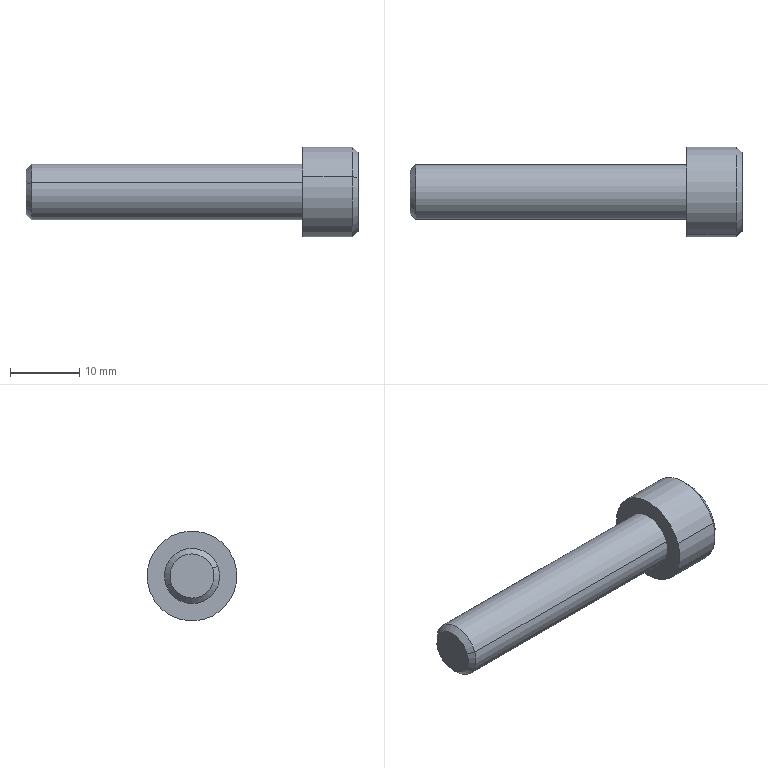Component | SolidWorks | LD101-02-HexagonScrew-M8X40-2-2 | 1 solid | 25 faces | box 48 x 13 x 13 mm | volume 2920 mm3 | plane 15 | cone 6 | cylinder 4 | commonest cylinder face diameters 13 x2 8 x2
STEP:
#1=COLOUR_RGB('',0.7922,0.8196,0.9333);
#2=FILL_AREA_STYLE_COLOUR('',#1);
#3=FILL_AREA_STYLE('',(#2));
#4=SURFACE_STYLE_FILL_AREA(#3);
#5=SURFACE_SIDE_STYLE('',(#4));
#6=SURFACE_STYLE_USAGE(.BOTH.,#5);
#7=PRESENTATION_STYLE_ASSIGNMENT((#6));
#8=CARTESIAN_POINT('',(13.374,-8.5,0.2505));
#9=VERTEX_POINT('',#8);
#10=CARTESIAN_POINT('',(13.374,-8.264,0.1634));
#11=VERTEX_POINT('',#10);
#12=CARTESIAN_POINT('',(13.374,-8.382,0.207));
#13=DIRECTION('',(-1.,0.,0.));
#14=DIRECTION('',(0.,-0.9384,0.3455));
#15=AXIS2_PLACEMENT_3D('',#12,#13,#14);
#16=CIRCLE('',#15,0.126);
#17=EDGE_CURVE('',#9,#11,#16,.T.);
#18=ORIENTED_EDGE('',*,*,#17,.F.);
#19=CARTESIAN_POINT('',(13.406,-8.53,0.2614));
#20=VERTEX_POINT('',#19);
#21=CARTESIAN_POINT('',(13.374,-8.5,0.2505));
#22=DIRECTION('',(0.7071,-0.6636,0.2443));
#23=VECTOR('',#22,39.37);
#24=LINE('',#21,#23);
#25=EDGE_CURVE('',#9,#20,#24,.T.);
#26=ORIENTED_EDGE('',*,*,#25,.T.);
#27=CARTESIAN_POINT('',(13.406,-8.234,0.1525));
#28=VERTEX_POINT('',#27);
#29=CARTESIAN_POINT('',(13.406,-8.382,0.207));
#30=DIRECTION('',(1.,-0.,-0.));
#31=DIRECTION('',(0.,-0.9384,0.3455));
#32=AXIS2_PLACEMENT_3D('',#29,#30,#31);
#33=CIRCLE('',#32,0.1575);
#34=EDGE_CURVE('',#28,#20,#33,.T.);
#35=ORIENTED_EDGE('',*,*,#34,.F.);
#36=CARTESIAN_POINT('',(13.374,-8.264,0.1634));
#37=DIRECTION('',(0.7071,0.6636,-0.2443));
#38=VECTOR('',#37,39.37);
#39=LINE('',#36,#38);
#40=EDGE_CURVE('',#11,#28,#39,.T.);
#41=ORIENTED_EDGE('',*,*,#40,.F.);
#42=EDGE_LOOP('',(#18,#26,#35,#41));
#43=FACE_OUTER_BOUND('',#42,.T.);
#44=CARTESIAN_POINT('',(13.374,-8.382,0.207));
#45=DIRECTION('',(1.,-0.,-0.));
#46=DIRECTION('',(0.,0.9384,-0.3455));
#47=AXIS2_PLACEMENT_3D('',#44,#45,#46);
#48=CONICAL_SURFACE('',#47,0.126,0.7854);
#49=ADVANCED_FACE('',(#43),#48,.T.);
#50=CARTESIAN_POINT('',(15.233,-8.622,0.2954));
#51=VERTEX_POINT('',#50);
#52=CARTESIAN_POINT('',(15.233,-8.142,0.1185));
#53=VERTEX_POINT('',#52);
#54=CARTESIAN_POINT('',(15.233,-8.382,0.207));
#55=DIRECTION('',(-1.,0.,0.));
#56=DIRECTION('',(0.,-0.9384,0.3455));
#57=AXIS2_PLACEMENT_3D('',#54,#55,#56);
#58=CIRCLE('',#57,0.2559);
#59=EDGE_CURVE('',#51,#53,#58,.T.);
#60=ORIENTED_EDGE('',*,*,#59,.T.);
#61=CARTESIAN_POINT('',(14.949,-8.142,0.1185));
#62=VERTEX_POINT('',#61);
#63=CARTESIAN_POINT('',(15.091,-8.142,0.1185));
#64=DIRECTION('',(-1.,0.,0.));
#65=VECTOR('',#64,39.37);
#66=LINE('',#63,#65);
#67=EDGE_CURVE('',#53,#62,#66,.T.);
#68=ORIENTED_EDGE('',*,*,#67,.T.);
#69=CARTESIAN_POINT('',(14.949,-8.622,0.2954));
#70=VERTEX_POINT('',#69);
#71=CARTESIAN_POINT('',(14.949,-8.382,0.207));
#72=DIRECTION('',(1.,-0.,-0.));
#73=DIRECTION('',(0.,-0.9384,0.3455));
#74=AXIS2_PLACEMENT_3D('',#71,#72,#73);
#75=CIRCLE('',#74,0.2559);
#76=EDGE_CURVE('',#62,#70,#75,.T.);
#77=ORIENTED_EDGE('',*,*,#76,.T.);
#78=CARTESIAN_POINT('',(15.091,-8.622,0.2954));
#79=DIRECTION('',(-1.,0.,0.));
#80=VECTOR('',#79,39.37);
#81=LINE('',#78,#80);
#82=EDGE_CURVE('',#51,#70,#81,.T.);
#83=ORIENTED_EDGE('',*,*,#82,.F.);
#84=EDGE_LOOP('',(#60,#68,#77,#83));
#85=FACE_OUTER_BOUND('',#84,.T.);
#86=CARTESIAN_POINT('',(15.091,-8.382,0.207));
#87=DIRECTION('',(-1.,0.,0.));
#88=DIRECTION('',(0.,-0.9384,0.3455));
#89=AXIS2_PLACEMENT_3D('',#86,#87,#88);
#90=CYLINDRICAL_SURFACE('',#89,0.2559);
#91=ADVANCED_FACE('',(#85),#90,.T.);
#92=CARTESIAN_POINT('',(15.264,-8.592,0.2845));
#93=VERTEX_POINT('',#92);
#94=CARTESIAN_POINT('',(15.264,-8.171,0.1294));
#95=VERTEX_POINT('',#94);
#96=CARTESIAN_POINT('',(15.264,-8.382,0.207));
#97=DIRECTION('',(-1.,0.,0.));
#98=DIRECTION('',(0.,-0.9384,0.3455));
#99=AXIS2_PLACEMENT_3D('',#96,#97,#98);
#100=CIRCLE('',#99,0.2244);
#101=EDGE_CURVE('',#93,#95,#100,.T.);
#102=ORIENTED_EDGE('',*,*,#101,.T.);
#103=CARTESIAN_POINT('',(15.233,-8.142,0.1185));
#104=DIRECTION('',(-0.7071,0.6636,-0.2443));
#105=VECTOR('',#104,39.37);
#106=LINE('',#103,#105);
#107=EDGE_CURVE('',#95,#53,#106,.T.);
#108=ORIENTED_EDGE('',*,*,#107,.T.);
#109=ORIENTED_EDGE('',*,*,#59,.F.);
#110=CARTESIAN_POINT('',(15.233,-8.622,0.2954));
#111=DIRECTION('',(-0.7071,-0.6636,0.2443));
#112=VECTOR('',#111,39.37);
#113=LINE('',#110,#112);
#114=EDGE_CURVE('',#93,#51,#113,.T.);
#115=ORIENTED_EDGE('',*,*,#114,.F.);
#116=EDGE_LOOP('',(#102,#108,#109,#115));
#117=FACE_OUTER_BOUND('',#116,.T.);
#118=CARTESIAN_POINT('',(15.233,-8.382,0.207));
#119=DIRECTION('',(-1.,0.,0.));
#120=DIRECTION('',(0.,-0.9384,0.3455));
#121=AXIS2_PLACEMENT_3D('',#118,#119,#120);
#122=CONICAL_SURFACE('',#121,0.2559,0.7854);
#123=ADVANCED_FACE('',(#117),#122,.T.);
#124=CARTESIAN_POINT('',(14.949,-8.234,0.1525));
#125=VERTEX_POINT('',#124);
#126=CARTESIAN_POINT('',(14.949,-8.53,0.2614));
#127=VERTEX_POINT('',#126);
#128=CARTESIAN_POINT('',(14.949,-8.382,0.207));
#129=DIRECTION('',(1.,-0.,-0.));
#130=DIRECTION('',(0.,-0.9384,0.3455));
#131=AXIS2_PLACEMENT_3D('',#128,#129,#130);
#132=CIRCLE('',#131,0.1575);
#133=EDGE_CURVE('',#125,#127,#132,.T.);
#134=ORIENTED_EDGE('',*,*,#133,.F.);
#135=CARTESIAN_POINT('',(14.767,-8.234,0.1525));
#136=DIRECTION('',(-1.,0.,0.));
#137=VECTOR('',#136,39.37);
#138=LINE('',#135,#137);
#139=EDGE_CURVE('',#125,#28,#138,.T.);
#140=ORIENTED_EDGE('',*,*,#139,.T.);
#141=ORIENTED_EDGE('',*,*,#34,.T.);
#142=CARTESIAN_POINT('',(14.767,-8.53,0.2614));
#143=DIRECTION('',(-1.,0.,0.));
#144=VECTOR('',#143,39.37);
#145=LINE('',#142,#144);
#146=EDGE_CURVE('',#127,#20,#145,.T.);
#147=ORIENTED_EDGE('',*,*,#146,.F.);
#148=EDGE_LOOP('',(#134,#140,#141,#147));
#149=FACE_OUTER_BOUND('',#148,.T.);
#150=CARTESIAN_POINT('',(14.767,-8.382,0.207));
#151=DIRECTION('',(-1.,0.,0.));
#152=DIRECTION('',(0.,-0.9384,0.3455));
#153=AXIS2_PLACEMENT_3D('',#150,#151,#152);
#154=CYLINDRICAL_SURFACE('',#153,0.1575);
#155=ADVANCED_FACE('',(#149),#154,.T.);
#156=CARTESIAN_POINT('',(15.075,-8.382,0.207));
#157=VERTEX_POINT('',#156);
#158=CARTESIAN_POINT('',(15.107,-8.271,0.1661));
#159=VERTEX_POINT('',#158);
#160=CARTESIAN_POINT('',(15.107,-8.271,0.1661));
#161=DIRECTION('',(0.2588,0.9064,-0.3338));
#162=VECTOR('',#161,39.37);
#163=LINE('',#160,#162);
#164=EDGE_CURVE('',#157,#159,#163,.T.);
#165=ORIENTED_EDGE('',*,*,#164,.F.);
#166=CARTESIAN_POINT('',(15.107,-8.493,0.2478));
#167=VERTEX_POINT('',#166);
#168=CARTESIAN_POINT('',(15.107,-8.493,0.2478));
#169=DIRECTION('',(0.2588,-0.9064,0.3338));
#170=VECTOR('',#169,39.37);
#171=LINE('',#168,#170);
#172=EDGE_CURVE('',#157,#167,#171,.T.);
#173=ORIENTED_EDGE('',*,*,#172,.T.);
#174=CARTESIAN_POINT('',(15.107,-8.473,0.1314));
#175=VERTEX_POINT('',#174);
#176=CARTESIAN_POINT('',(15.107,-8.382,0.207));
#177=DIRECTION('',(-1.,0.,0.));
#178=DIRECTION('',(0.,0.9384,-0.3455));
#179=AXIS2_PLACEMENT_3D('',#176,#177,#178);
#180=CIRCLE('',#179,0.1181);
#181=EDGE_CURVE('',#175,#167,#180,.T.);
#182=ORIENTED_EDGE('',*,*,#181,.F.);
#183=CARTESIAN_POINT('',(15.107,-8.362,0.09056));
#184=VERTEX_POINT('',#183);
#185=CARTESIAN_POINT('',(15.107,-8.382,0.207));
#186=DIRECTION('',(-1.,0.,0.));
#187=DIRECTION('',(0.,0.9384,-0.3455));
#188=AXIS2_PLACEMENT_3D('',#185,#186,#187);
#189=CIRCLE('',#188,0.1181);
#190=EDGE_CURVE('',#184,#175,#189,.T.);
#191=ORIENTED_EDGE('',*,*,#190,.F.);
#192=CARTESIAN_POINT('',(15.107,-8.382,0.207));
#193=DIRECTION('',(1.,-0.,-0.));
#194=DIRECTION('',(0.,0.9384,-0.3455));
#195=AXIS2_PLACEMENT_3D('',#192,#193,#194);
#196=CIRCLE('',#195,0.1181);
#197=EDGE_CURVE('',#184,#159,#196,.T.);
#198=ORIENTED_EDGE('',*,*,#197,.T.);
#199=EDGE_LOOP('',(#165,#173,#182,#191,#198));
#200=FACE_OUTER_BOUND('',#199,.T.);
#201=CARTESIAN_POINT('',(15.107,-8.382,0.207));
#202=DIRECTION('',(1.,-0.,-0.));
#203=DIRECTION('',(0.,0.9384,-0.3455));
#204=AXIS2_PLACEMENT_3D('',#201,#202,#203);
#205=CONICAL_SURFACE('',#204,0.1181,1.309);
#206=ADVANCED_FACE('',(#200),#205,.F.);
#207=ORIENTED_EDGE('',*,*,#67,.F.);
#208=CARTESIAN_POINT('',(15.233,-8.382,0.207));
#209=DIRECTION('',(-1.,0.,0.));
#210=DIRECTION('',(0.,-0.9384,0.3455));
#211=AXIS2_PLACEMENT_3D('',#208,#209,#210);
#212=CIRCLE('',#211,0.2559);
#213=EDGE_CURVE('',#53,#51,#212,.T.);
#214=ORIENTED_EDGE('',*,*,#213,.T.);
#215=ORIENTED_EDGE('',*,*,#82,.T.);
#216=CARTESIAN_POINT('',(14.949,-8.382,0.207));
#217=DIRECTION('',(1.,-0.,-0.));
#218=DIRECTION('',(0.,-0.9384,0.3455));
#219=AXIS2_PLACEMENT_3D('',#216,#217,#218);
#220=CIRCLE('',#219,0.2559);
#221=EDGE_CURVE('',#70,#62,#220,.T.);
#222=ORIENTED_EDGE('',*,*,#221,.T.);
#223=EDGE_LOOP('',(#207,#214,#215,#222));
#224=FACE_OUTER_BOUND('',#223,.T.);
#225=CARTESIAN_POINT('',(15.091,-8.382,0.207));
#226=DIRECTION('',(-1.,0.,0.));
#227=DIRECTION('',(0.,-0.9384,0.3455));
#228=AXIS2_PLACEMENT_3D('',#225,#226,#227);
#229=CYLINDRICAL_SURFACE('',#228,0.2559);
#230=ADVANCED_FACE('',(#224),#229,.T.);
#231=ORIENTED_EDGE('',*,*,#107,.F.);
#232=CARTESIAN_POINT('',(15.264,-8.382,0.207));
#233=DIRECTION('',(-1.,0.,0.));
#234=DIRECTION('',(0.,-0.9384,0.3455));
#235=AXIS2_PLACEMENT_3D('',#232,#233,#234);
#236=CIRCLE('',#235,0.2244);
#237=EDGE_CURVE('',#95,#93,#236,.T.);
#238=ORIENTED_EDGE('',*,*,#237,.T.);
#239=ORIENTED_EDGE('',*,*,#114,.T.);
#240=ORIENTED_EDGE('',*,*,#213,.F.);
#241=EDGE_LOOP('',(#231,#238,#239,#240));
#242=FACE_OUTER_BOUND('',#241,.T.);
#243=CARTESIAN_POINT('',(15.233,-8.382,0.207));
#244=DIRECTION('',(-1.,0.,0.));
#245=DIRECTION('',(0.,-0.9384,0.3455));
#246=AXIS2_PLACEMENT_3D('',#243,#244,#245);
#247=CONICAL_SURFACE('',#246,0.2559,0.7854);
#248=ADVANCED_FACE('',(#242),#247,.T.);
#249=CARTESIAN_POINT('',(14.949,-8.382,0.207));
#250=DIRECTION('',(1.,-0.,-0.));
#251=DIRECTION('',(0.,-0.9384,0.3455));
#252=AXIS2_PLACEMENT_3D('',#249,#250,#251);
#253=CIRCLE('',#252,0.1575);
#254=EDGE_CURVE('',#127,#125,#253,.T.);
#255=ORIENTED_EDGE('',*,*,#254,.T.);
#256=ORIENTED_EDGE('',*,*,#133,.T.);
#257=EDGE_LOOP('',(#255,#256));
#258=FACE_BOUND('',#257,.T.);
#259=ORIENTED_EDGE('',*,*,#221,.F.);
#260=ORIENTED_EDGE('',*,*,#76,.F.);
#261=EDGE_LOOP('',(#259,#260));
#262=FACE_OUTER_BOUND('',#261,.T.);
#263=CARTESIAN_POINT('',(14.949,-8.31,0.4009));
#264=DIRECTION('',(-1.,0.,0.));
#265=DIRECTION('',(-0.,-0.9384,0.3455));
#266=AXIS2_PLACEMENT_3D('',#263,#264,#265);
#267=PLANE('',#266);
#268=ADVANCED_FACE('',(#258,#262),#267,.T.);
#269=ORIENTED_EDGE('',*,*,#101,.F.);
#270=ORIENTED_EDGE('',*,*,#237,.F.);
#271=EDGE_LOOP('',(#269,#270));
#272=FACE_OUTER_BOUND('',#271,.T.);
#273=CARTESIAN_POINT('',(15.264,-8.469,0.3118));
#274=VERTEX_POINT('',#273);
#275=CARTESIAN_POINT('',(15.264,-8.335,0.3349));
#276=VERTEX_POINT('',#275);
#277=CARTESIAN_POINT('',(15.264,-8.469,0.3118));
#278=DIRECTION('',(0.,0.9855,0.17));
#279=VECTOR('',#278,39.37);
#280=LINE('',#277,#279);
#281=EDGE_CURVE('',#274,#276,#280,.T.);
#282=ORIENTED_EDGE('',*,*,#281,.T.);
#283=CARTESIAN_POINT('',(15.264,-8.247,0.2301));
#284=VERTEX_POINT('',#283);
#285=CARTESIAN_POINT('',(15.264,-8.335,0.3349));
#286=DIRECTION('',(0.,0.6399,-0.7684));
#287=VECTOR('',#286,39.37);
#288=LINE('',#285,#287);
#289=EDGE_CURVE('',#276,#284,#288,.T.);
#290=ORIENTED_EDGE('',*,*,#289,.T.);
#291=CARTESIAN_POINT('',(15.264,-8.294,0.1022));
#292=VERTEX_POINT('',#291);
#293=CARTESIAN_POINT('',(15.264,-8.232,0.2714));
#294=DIRECTION('',(-0.,-0.3455,-0.9384));
#295=VECTOR('',#294,39.37);
#296=LINE('',#293,#295);
#297=EDGE_CURVE('',#284,#292,#296,.T.);
#298=ORIENTED_EDGE('',*,*,#297,.T.);
#299=CARTESIAN_POINT('',(15.264,-8.429,0.07897));
#300=VERTEX_POINT('',#299);
#301=CARTESIAN_POINT('',(15.264,-8.294,0.1022));
#302=DIRECTION('',(-0.,-0.9855,-0.17));
#303=VECTOR('',#302,39.37);
#304=LINE('',#301,#303);
#305=EDGE_CURVE('',#292,#300,#304,.T.);
#306=ORIENTED_EDGE('',*,*,#305,.T.);
#307=CARTESIAN_POINT('',(15.264,-8.516,0.1838));
#308=VERTEX_POINT('',#307);
#309=CARTESIAN_POINT('',(15.264,-8.429,0.07897));
#310=DIRECTION('',(-0.,-0.6399,0.7684));
#311=VECTOR('',#310,39.37);
#312=LINE('',#309,#311);
#313=EDGE_CURVE('',#300,#308,#312,.T.);
#314=ORIENTED_EDGE('',*,*,#313,.T.);
#315=CARTESIAN_POINT('',(15.264,-8.454,0.3531));
#316=DIRECTION('',(0.,0.3455,0.9384));
#317=VECTOR('',#316,39.37);
#318=LINE('',#315,#317);
#319=EDGE_CURVE('',#308,#274,#318,.T.);
#320=ORIENTED_EDGE('',*,*,#319,.T.);
#321=EDGE_LOOP('',(#282,#290,#298,#306,#314,#320));
#322=FACE_BOUND('',#321,.T.);
#323=CARTESIAN_POINT('',(15.264,-8.343,0.3122));
#324=DIRECTION('',(1.,-0.,-0.));
#325=DIRECTION('',(0.,0.9384,-0.3455));
#326=AXIS2_PLACEMENT_3D('',#323,#324,#325);
#327=PLANE('',#326);
#328=ADVANCED_FACE('',(#272,#322),#327,.T.);
#329=ORIENTED_EDGE('',*,*,#139,.F.);
#330=ORIENTED_EDGE('',*,*,#254,.F.);
#331=ORIENTED_EDGE('',*,*,#146,.T.);
#332=CARTESIAN_POINT('',(13.406,-8.382,0.207));
#333=DIRECTION('',(1.,-0.,-0.));
#334=DIRECTION('',(0.,-0.9384,0.3455));
#335=AXIS2_PLACEMENT_3D('',#332,#333,#334);
#336=CIRCLE('',#335,0.1575);
#337=EDGE_CURVE('',#20,#28,#336,.T.);
#338=ORIENTED_EDGE('',*,*,#337,.T.);
#339=EDGE_LOOP('',(#329,#330,#331,#338));
#340=FACE_OUTER_BOUND('',#339,.T.);
#341=CARTESIAN_POINT('',(14.767,-8.382,0.207));
#342=DIRECTION('',(-1.,0.,0.));
#343=DIRECTION('',(0.,-0.9384,0.3455));
#344=AXIS2_PLACEMENT_3D('',#341,#342,#343);
#345=CYLINDRICAL_SURFACE('',#344,0.1575);
#346=ADVANCED_FACE('',(#340),#345,.T.);
#347=CARTESIAN_POINT('',(15.107,-8.335,0.3349));
#348=VERTEX_POINT('',#347);
#349=CARTESIAN_POINT('',(15.264,-8.335,0.3349));
#350=DIRECTION('',(1.,-0.,-0.));
#351=VECTOR('',#350,39.37);
#352=LINE('',#349,#351);
#353=EDGE_CURVE('',#348,#276,#352,.T.);
#354=ORIENTED_EDGE('',*,*,#353,.F.);
#355=CARTESIAN_POINT('',(15.107,-8.291,0.2825));
#356=VERTEX_POINT('',#355);
#357=CARTESIAN_POINT('',(15.107,-8.247,0.2301));
#358=DIRECTION('',(-0.,-0.6399,0.7684));
#359=VECTOR('',#358,39.37);
#360=LINE('',#357,#359);
#361=EDGE_CURVE('',#356,#348,#360,.T.);
#362=ORIENTED_EDGE('',*,*,#361,.F.);
#363=CARTESIAN_POINT('',(15.107,-8.247,0.2301));
#364=VERTEX_POINT('',#363);
#365=CARTESIAN_POINT('',(15.107,-8.291,0.2825));
#366=DIRECTION('',(0.,0.6399,-0.7684));
#367=VECTOR('',#366,39.37);
#368=LINE('',#365,#367);
#369=EDGE_CURVE('',#356,#364,#368,.T.);
#370=ORIENTED_EDGE('',*,*,#369,.T.);
#371=CARTESIAN_POINT('',(15.264,-8.247,0.2301));
#372=DIRECTION('',(-1.,0.,0.));
#373=VECTOR('',#372,39.37);
#374=LINE('',#371,#373);
#375=EDGE_CURVE('',#284,#364,#374,.T.);
#376=ORIENTED_EDGE('',*,*,#375,.F.);
#377=ORIENTED_EDGE('',*,*,#289,.F.);
#378=EDGE_LOOP('',(#354,#362,#370,#376,#377));
#379=FACE_OUTER_BOUND('',#378,.T.);
#380=CARTESIAN_POINT('',(15.264,-8.247,0.2301));
#381=DIRECTION('',(0.,0.7684,0.6399));
#382=DIRECTION('',(0.,0.6399,-0.7684));
#383=AXIS2_PLACEMENT_3D('',#380,#381,#382);
#384=PLANE('',#383);
#385=ADVANCED_FACE('',(#379),#384,.F.);
#386=CARTESIAN_POINT('',(15.107,-8.469,0.3118));
#387=VERTEX_POINT('',#386);
#388=CARTESIAN_POINT('',(15.264,-8.469,0.3118));
#389=DIRECTION('',(1.,-0.,-0.));
#390=VECTOR('',#389,39.37);
#391=LINE('',#388,#390);
#392=EDGE_CURVE('',#387,#274,#391,.T.);
#393=ORIENTED_EDGE('',*,*,#392,.F.);
#394=CARTESIAN_POINT('',(15.107,-8.402,0.3233));
#395=VERTEX_POINT('',#394);
#396=CARTESIAN_POINT('',(15.107,-8.469,0.3118));
#397=DIRECTION('',(0.,0.9855,0.17));
#398=VECTOR('',#397,39.37);
#399=LINE('',#396,#398);
#400=EDGE_CURVE('',#387,#395,#399,.T.);
#401=ORIENTED_EDGE('',*,*,#400,.T.);
#402=CARTESIAN_POINT('',(15.107,-8.335,0.3349));
#403=DIRECTION('',(-0.,-0.9855,-0.17));
#404=VECTOR('',#403,39.37);
#405=LINE('',#402,#404);
#406=EDGE_CURVE('',#348,#395,#405,.T.);
#407=ORIENTED_EDGE('',*,*,#406,.F.);
#408=ORIENTED_EDGE('',*,*,#353,.T.);
#409=ORIENTED_EDGE('',*,*,#281,.F.);
#410=EDGE_LOOP('',(#393,#401,#407,#408,#409));
#411=FACE_OUTER_BOUND('',#410,.T.);
#412=CARTESIAN_POINT('',(15.264,-8.335,0.3349));
#413=DIRECTION('',(-0.,-0.17,0.9855));
#414=DIRECTION('',(0.,0.9855,0.17));
#415=AXIS2_PLACEMENT_3D('',#412,#413,#414);
#416=PLANE('',#415);
#417=ADVANCED_FACE('',(#411),#416,.F.);
#418=CARTESIAN_POINT('',(15.107,-8.516,0.1838));
#419=VERTEX_POINT('',#418);
#420=CARTESIAN_POINT('',(15.264,-8.516,0.1838));
#421=DIRECTION('',(1.,-0.,-0.));
#422=VECTOR('',#421,39.37);
#423=LINE('',#420,#422);
#424=EDGE_CURVE('',#419,#308,#423,.T.);
#425=ORIENTED_EDGE('',*,*,#424,.F.);
#426=CARTESIAN_POINT('',(15.107,-8.493,0.2478));
#427=DIRECTION('',(0.,0.3455,0.9384));
#428=VECTOR('',#427,39.37);
#429=LINE('',#426,#428);
#430=EDGE_CURVE('',#419,#167,#429,.T.);
#431=ORIENTED_EDGE('',*,*,#430,.T.);
#432=CARTESIAN_POINT('',(15.107,-8.493,0.2478));
#433=DIRECTION('',(0.,0.3455,0.9384));
#434=VECTOR('',#433,39.37);
#435=LINE('',#432,#434);
#436=EDGE_CURVE('',#167,#387,#435,.T.);
#437=ORIENTED_EDGE('',*,*,#436,.T.);
#438=ORIENTED_EDGE('',*,*,#392,.T.);
#439=ORIENTED_EDGE('',*,*,#319,.F.);
#440=EDGE_LOOP('',(#425,#431,#437,#438,#439));
#441=FACE_OUTER_BOUND('',#440,.T.);
#442=CARTESIAN_POINT('',(15.264,-8.469,0.3118));
#443=DIRECTION('',(-0.,-0.9384,0.3455));
#444=DIRECTION('',(1.,-0.,-0.));
#445=AXIS2_PLACEMENT_3D('',#442,#443,#444);
#446=PLANE('',#445);
#447=ADVANCED_FACE('',(#441),#446,.F.);
#448=CARTESIAN_POINT('',(15.107,-8.429,0.07897));
#449=VERTEX_POINT('',#448);
#450=CARTESIAN_POINT('',(15.264,-8.429,0.07897));
#451=DIRECTION('',(1.,-0.,-0.));
#452=VECTOR('',#451,39.37);
#453=LINE('',#450,#452);
#454=EDGE_CURVE('',#449,#300,#453,.T.);
#455=ORIENTED_EDGE('',*,*,#454,.F.);
#456=CARTESIAN_POINT('',(15.107,-8.516,0.1838));
#457=DIRECTION('',(0.,0.6399,-0.7684));
#458=VECTOR('',#457,39.37);
#459=LINE('',#456,#458);
#460=EDGE_CURVE('',#175,#449,#459,.T.);
#461=ORIENTED_EDGE('',*,*,#460,.F.);
#462=CARTESIAN_POINT('',(15.107,-8.473,0.1314));
#463=DIRECTION('',(-0.,-0.6399,0.7684));
#464=VECTOR('',#463,39.37);
#465=LINE('',#462,#464);
#466=EDGE_CURVE('',#175,#419,#465,.T.);
#467=ORIENTED_EDGE('',*,*,#466,.T.);
#468=ORIENTED_EDGE('',*,*,#424,.T.);
#469=ORIENTED_EDGE('',*,*,#313,.F.);
#470=EDGE_LOOP('',(#455,#461,#467,#468,#469));
#471=FACE_OUTER_BOUND('',#470,.T.);
#472=CARTESIAN_POINT('',(15.264,-8.516,0.1838));
#473=DIRECTION('',(-0.,-0.7684,-0.6399));
#474=DIRECTION('',(-0.,-0.6399,0.7684));
#475=AXIS2_PLACEMENT_3D('',#472,#473,#474);
#476=PLANE('',#475);
#477=ADVANCED_FACE('',(#471),#476,.F.);
#478=CARTESIAN_POINT('',(15.107,-8.294,0.1022));
#479=VERTEX_POINT('',#478);
#480=CARTESIAN_POINT('',(15.264,-8.294,0.1022));
#481=DIRECTION('',(1.,-0.,-0.));
#482=VECTOR('',#481,39.37);
#483=LINE('',#480,#482);
#484=EDGE_CURVE('',#479,#292,#483,.T.);
#485=ORIENTED_EDGE('',*,*,#484,.F.);
#486=CARTESIAN_POINT('',(15.107,-8.429,0.07897));
#487=DIRECTION('',(0.,0.9855,0.17));
#488=VECTOR('',#487,39.37);
#489=LINE('',#486,#488);
#490=EDGE_CURVE('',#184,#479,#489,.T.);
#491=ORIENTED_EDGE('',*,*,#490,.F.);
#492=CARTESIAN_POINT('',(15.107,-8.429,0.07897));
#493=DIRECTION('',(0.,0.9855,0.17));
#494=VECTOR('',#493,39.37);
#495=LINE('',#492,#494);
#496=EDGE_CURVE('',#449,#184,#495,.T.);
#497=ORIENTED_EDGE('',*,*,#496,.F.);
#498=ORIENTED_EDGE('',*,*,#454,.T.);
#499=ORIENTED_EDGE('',*,*,#305,.F.);
#500=EDGE_LOOP('',(#485,#491,#497,#498,#499));
#501=FACE_OUTER_BOUND('',#500,.T.);
#502=CARTESIAN_POINT('',(15.264,-8.429,0.07897));
#503=DIRECTION('',(0.,0.17,-0.9855));
#504=DIRECTION('',(-0.,-0.9855,-0.17));
#505=AXIS2_PLACEMENT_3D('',#502,#503,#504);
#506=PLANE('',#505);
#507=ADVANCED_FACE('',(#501),#506,.F.);
#508=ORIENTED_EDGE('',*,*,#375,.T.);
#509=CARTESIAN_POINT('',(15.107,-8.271,0.1661));
#510=DIRECTION('',(-0.,-0.3455,-0.9384));
#511=VECTOR('',#510,39.37);
#512=LINE('',#509,#511);
#513=EDGE_CURVE('',#364,#159,#512,.T.);
#514=ORIENTED_EDGE('',*,*,#513,.T.);
#515=CARTESIAN_POINT('',(15.107,-8.294,0.1022));
#516=DIRECTION('',(0.,0.3455,0.9384));
#517=VECTOR('',#516,39.37);
#518=LINE('',#515,#517);
#519=EDGE_CURVE('',#479,#159,#518,.T.);
#520=ORIENTED_EDGE('',*,*,#519,.F.);
#521=ORIENTED_EDGE('',*,*,#484,.T.);
#522=ORIENTED_EDGE('',*,*,#297,.F.);
#523=EDGE_LOOP('',(#508,#514,#520,#521,#522));
#524=FACE_OUTER_BOUND('',#523,.T.);
#525=CARTESIAN_POINT('',(15.264,-8.294,0.1022));
#526=DIRECTION('',(0.,0.9384,-0.3455));
#527=DIRECTION('',(-1.,0.,0.));
#528=AXIS2_PLACEMENT_3D('',#525,#526,#527);
#529=PLANE('',#528);
#530=ADVANCED_FACE('',(#524),#529,.F.);
#531=ORIENTED_EDGE('',*,*,#361,.T.);
#532=ORIENTED_EDGE('',*,*,#406,.T.);
#533=CARTESIAN_POINT('',(15.107,-8.382,0.207));
#534=DIRECTION('',(-1.,0.,0.));
#535=DIRECTION('',(0.,0.9384,-0.3455));
#536=AXIS2_PLACEMENT_3D('',#533,#534,#535);
#537=CIRCLE('',#536,0.1181);
#538=EDGE_CURVE('',#395,#356,#537,.T.);
#539=ORIENTED_EDGE('',*,*,#538,.T.);
#540=EDGE_LOOP('',(#531,#532,#539));
#541=FACE_OUTER_BOUND('',#540,.T.);
#542=CARTESIAN_POINT('',(15.107,-8.382,0.207));
#543=DIRECTION('',(-1.,0.,0.));
#544=DIRECTION('',(-0.,-0.9384,0.3455));
#545=AXIS2_PLACEMENT_3D('',#542,#543,#544);
#546=PLANE('',#545);
#547=ADVANCED_FACE('',(#541),#546,.F.);
#548=ORIENTED_EDGE('',*,*,#460,.T.);
#549=ORIENTED_EDGE('',*,*,#496,.T.);
#550=ORIENTED_EDGE('',*,*,#190,.T.);
#551=EDGE_LOOP('',(#548,#549,#550));
#552=FACE_OUTER_BOUND('',#551,.T.);
#553=CARTESIAN_POINT('',(15.107,-8.382,0.207));
#554=DIRECTION('',(-1.,0.,0.));
#555=DIRECTION('',(-0.,-0.9384,0.3455));
#556=AXIS2_PLACEMENT_3D('',#553,#554,#555);
#557=PLANE('',#556);
#558=ADVANCED_FACE('',(#552),#557,.F.);
#559=ORIENTED_EDGE('',*,*,#490,.T.);
#560=ORIENTED_EDGE('',*,*,#519,.T.);
#561=ORIENTED_EDGE('',*,*,#197,.F.);
#562=EDGE_LOOP('',(#559,#560,#561));
#563=FACE_OUTER_BOUND('',#562,.T.);
#564=CARTESIAN_POINT('',(15.107,-8.382,0.207));
#565=DIRECTION('',(-1.,0.,0.));
#566=DIRECTION('',(-0.,-0.9384,0.3455));
#567=AXIS2_PLACEMENT_3D('',#564,#565,#566);
#568=PLANE('',#567);
#569=ADVANCED_FACE('',(#563),#568,.F.);
#570=ORIENTED_EDGE('',*,*,#172,.F.);
#571=ORIENTED_EDGE('',*,*,#164,.T.);
#572=CARTESIAN_POINT('',(15.107,-8.382,0.207));
#573=DIRECTION('',(-1.,0.,0.));
#574=DIRECTION('',(0.,0.9384,-0.3455));
#575=AXIS2_PLACEMENT_3D('',#572,#573,#574);
#576=CIRCLE('',#575,0.1181);
#577=EDGE_CURVE('',#356,#159,#576,.T.);
#578=ORIENTED_EDGE('',*,*,#577,.F.);
#579=ORIENTED_EDGE('',*,*,#538,.F.);
#580=CARTESIAN_POINT('',(15.107,-8.382,0.207));
#581=DIRECTION('',(-1.,0.,0.));
#582=DIRECTION('',(0.,0.9384,-0.3455));
#583=AXIS2_PLACEMENT_3D('',#580,#581,#582);
#584=CIRCLE('',#583,0.1181);
#585=EDGE_CURVE('',#167,#395,#584,.T.);
#586=ORIENTED_EDGE('',*,*,#585,.F.);
#587=EDGE_LOOP('',(#570,#571,#578,#579,#586));
#588=FACE_OUTER_BOUND('',#587,.T.);
#589=CARTESIAN_POINT('',(15.107,-8.382,0.207));
#590=DIRECTION('',(1.,-0.,-0.));
#591=DIRECTION('',(0.,0.9384,-0.3455));
#592=AXIS2_PLACEMENT_3D('',#589,#590,#591);
#593=CONICAL_SURFACE('',#592,0.1181,1.309);
#594=ADVANCED_FACE('',(#588),#593,.F.);
#595=ORIENTED_EDGE('',*,*,#513,.F.);
#596=ORIENTED_EDGE('',*,*,#369,.F.);
#597=ORIENTED_EDGE('',*,*,#577,.T.);
#598=EDGE_LOOP('',(#595,#596,#597));
#599=FACE_OUTER_BOUND('',#598,.T.);
#600=CARTESIAN_POINT('',(15.107,-8.382,0.207));
#601=DIRECTION('',(-1.,0.,0.));
#602=DIRECTION('',(-0.,-0.9384,0.3455));
#603=AXIS2_PLACEMENT_3D('',#600,#601,#602);
#604=PLANE('',#603);
#605=ADVANCED_FACE('',(#599),#604,.F.);
#606=ORIENTED_EDGE('',*,*,#400,.F.);
#607=ORIENTED_EDGE('',*,*,#436,.F.);
#608=ORIENTED_EDGE('',*,*,#585,.T.);
#609=EDGE_LOOP('',(#606,#607,#608));
#610=FACE_OUTER_BOUND('',#609,.T.);
#611=CARTESIAN_POINT('',(15.107,-8.382,0.207));
#612=DIRECTION('',(-1.,0.,0.));
#613=DIRECTION('',(-0.,-0.9384,0.3455));
#614=AXIS2_PLACEMENT_3D('',#611,#612,#613);
#615=PLANE('',#614);
#616=ADVANCED_FACE('',(#610),#615,.F.);
#617=ORIENTED_EDGE('',*,*,#430,.F.);
#618=ORIENTED_EDGE('',*,*,#466,.F.);
#619=ORIENTED_EDGE('',*,*,#181,.T.);
#620=EDGE_LOOP('',(#617,#618,#619));
#621=FACE_OUTER_BOUND('',#620,.T.);
#622=CARTESIAN_POINT('',(15.107,-8.382,0.207));
#623=DIRECTION('',(-1.,0.,0.));
#624=DIRECTION('',(-0.,-0.9384,0.3455));
#625=AXIS2_PLACEMENT_3D('',#622,#623,#624);
#626=PLANE('',#625);
#627=ADVANCED_FACE('',(#621),#626,.F.);
#628=CARTESIAN_POINT('',(13.374,-8.382,0.207));
#629=DIRECTION('',(-1.,0.,0.));
#630=DIRECTION('',(0.,-0.9384,0.3455));
#631=AXIS2_PLACEMENT_3D('',#628,#629,#630);
#632=CIRCLE('',#631,0.126);
#633=EDGE_CURVE('',#11,#9,#632,.T.);
#634=ORIENTED_EDGE('',*,*,#633,.T.);
#635=ORIENTED_EDGE('',*,*,#17,.T.);
#636=EDGE_LOOP('',(#634,#635));
#637=FACE_OUTER_BOUND('',#636,.T.);
#638=CARTESIAN_POINT('',(13.374,-8.382,0.207));
#639=DIRECTION('',(-1.,0.,0.));
#640=DIRECTION('',(-0.,-0.9384,0.3455));
#641=AXIS2_PLACEMENT_3D('',#638,#639,#640);
#642=PLANE('',#641);
#643=ADVANCED_FACE('',(#637),#642,.T.);
#644=ORIENTED_EDGE('',*,*,#25,.F.);
#645=ORIENTED_EDGE('',*,*,#633,.F.);
#646=ORIENTED_EDGE('',*,*,#40,.T.);
#647=ORIENTED_EDGE('',*,*,#337,.F.);
#648=EDGE_LOOP('',(#644,#645,#646,#647));
#649=FACE_OUTER_BOUND('',#648,.T.);
#650=CARTESIAN_POINT('',(13.374,-8.382,0.207));
#651=DIRECTION('',(1.,-0.,-0.));
#652=DIRECTION('',(0.,0.9384,-0.3455));
#653=AXIS2_PLACEMENT_3D('',#650,#651,#652);
#654=CONICAL_SURFACE('',#653,0.126,0.7854);
#655=ADVANCED_FACE('',(#649),#654,.T.);
#656=CLOSED_SHELL('',(#49,#91,#123,#155,#206,#230,#248,#268,#328,#346,#385,#417,#447,#477,#507,#530,#547,#558,#569,#594,#605,#616,#627,#643,#655));
#657=MANIFOLD_SOLID_BREP('',#656);
#658=STYLED_ITEM('',(#7),#657);
#659=(LENGTH_UNIT()NAMED_UNIT(*)SI_UNIT($,.METRE.));
#660=LENGTH_MEASURE_WITH_UNIT(LENGTH_MEASURE(0.0254),#659);
#661=DIMENSIONAL_EXPONENTS(1.,0.,0.,0.,0.,0.,0.);
#662=(CONVERSION_BASED_UNIT('',#660)LENGTH_UNIT()NAMED_UNIT(#661));
#663=UNCERTAINTY_MEASURE_WITH_UNIT(LENGTH_MEASURE(0.00001),#662,'','');
#664=(NAMED_UNIT(*)PLANE_ANGLE_UNIT()SI_UNIT($,.RADIAN.));
#665=(NAMED_UNIT(*)SI_UNIT($,.STERADIAN.)SOLID_ANGLE_UNIT());
#666=(GEOMETRIC_REPRESENTATION_CONTEXT(3)GLOBAL_UNCERTAINTY_ASSIGNED_CONTEXT((#663))GLOBAL_UNIT_ASSIGNED_CONTEXT((#662,#664,#665))REPRESENTATION_CONTEXT('',''));
#667=MECHANICAL_DESIGN_GEOMETRIC_PRESENTATION_REPRESENTATION('',(#658),#666);
#668=CARTESIAN_POINT('',(0.,0.,0.));
#669=DIRECTION('',(0.,0.,1.));
#670=DIRECTION('',(1.,0.,0.));
#671=AXIS2_PLACEMENT_3D('',#668,#669,#670);
#672=(LENGTH_UNIT()NAMED_UNIT(*)SI_UNIT($,.METRE.));
#673=LENGTH_MEASURE_WITH_UNIT(LENGTH_MEASURE(0.0254),#672);
#674=DIMENSIONAL_EXPONENTS(1.,0.,0.,0.,0.,0.,0.);
#675=(CONVERSION_BASED_UNIT('',#673)LENGTH_UNIT()NAMED_UNIT(#674));
#676=UNCERTAINTY_MEASURE_WITH_UNIT(LENGTH_MEASURE(0.00001),#675,'','');
#677=(NAMED_UNIT(*)PLANE_ANGLE_UNIT()SI_UNIT($,.RADIAN.));
#678=(NAMED_UNIT(*)SI_UNIT($,.STERADIAN.)SOLID_ANGLE_UNIT());
#679=(GEOMETRIC_REPRESENTATION_CONTEXT(3)GLOBAL_UNCERTAINTY_ASSIGNED_CONTEXT((#676))GLOBAL_UNIT_ASSIGNED_CONTEXT((#675,#677,#678))REPRESENTATION_CONTEXT('',''));
#680=ADVANCED_BREP_SHAPE_REPRESENTATION('',(#657,#671),#679);
#681=PRESENTATION_LAYER_ASSIGNMENT('','',(#658));